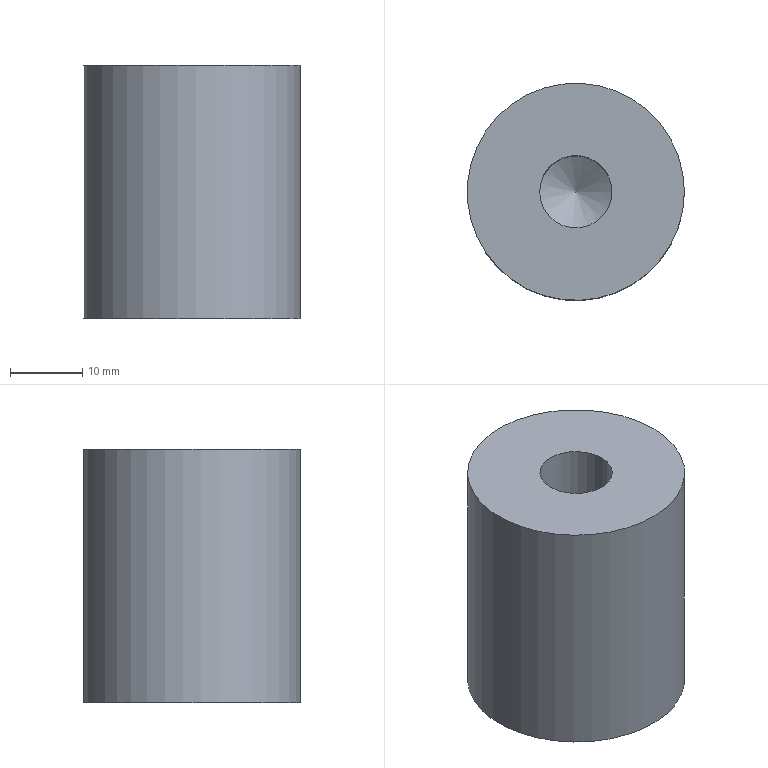Component | NX | CH3404_10-2 | 1 solid | 5 faces | box 30 x 30 x 35 mm | volume 22698 mm3 | cylinder 2 | plane 2 | cone 1 | commonest cylinder face diameters 30 x1 10 x1
STEP:
#1=CARTESIAN_POINT('',(0.,0.,0.));
#2=DIRECTION('',(0.,0.,1.));
#3=DIRECTION('',(1.,0.,0.));
#4=AXIS2_PLACEMENT_3D('',#1,#2,#3);
#5=CARTESIAN_POINT('',(15.,0.,146.));
#6=VERTEX_POINT('',#5);
#7=CARTESIAN_POINT('',(0.,0.,146.));
#8=DIRECTION('',(0.,0.,1.));
#9=DIRECTION('',(1.,0.,0.));
#10=AXIS2_PLACEMENT_3D('',#7,#8,#9);
#11=CIRCLE('',#10,15.);
#12=CARTESIAN_POINT('',(0.,0.,146.));
#13=DIRECTION('',(0.,0.,-1.));
#14=DIRECTION('',(-1.,0.,0.));
#15=AXIS2_PLACEMENT_3D('',#12,#13,#14);
#16=CYLINDRICAL_SURFACE('',#15,15.);
#17=CARTESIAN_POINT('',(9.425,0.));
#18=DIRECTION('',(-1.,0.));
#19=VECTOR('',#18,1.);
#20=LINE('',#17,#19);
#21=(GEOMETRIC_REPRESENTATION_CONTEXT(2)PARAMETRIC_REPRESENTATION_CONTEXT()REPRESENTATION_CONTEXT('',''));
#22=DEFINITIONAL_REPRESENTATION('',(#20),#21);
#23=PCURVE('',#16,#22);
#24=CARTESIAN_POINT('',(0.,0.,146.));
#25=DIRECTION('',(0.,0.,1.));
#26=DIRECTION('',(1.,0.,0.));
#27=AXIS2_PLACEMENT_3D('',#24,#25,#26);
#28=PLANE('',#27);
#29=CARTESIAN_POINT('',(0.,0.));
#30=DIRECTION('',(1.,0.));
#31=AXIS2_PLACEMENT_2D('',#29,#30);
#32=CIRCLE('',#31,15.);
#33=(GEOMETRIC_REPRESENTATION_CONTEXT(2)PARAMETRIC_REPRESENTATION_CONTEXT()REPRESENTATION_CONTEXT('',''));
#34=DEFINITIONAL_REPRESENTATION('',(#32),#33);
#35=PCURVE('',#28,#34);
#36=SURFACE_CURVE('',#11,(#23,#35),.PCURVE_S1.);
#37=EDGE_CURVE('',#6,#6,#36,.T.);
#38=ORIENTED_EDGE('',*,*,#37,.F.);
#39=CARTESIAN_POINT('',(15.,0.,111.));
#40=VERTEX_POINT('',#39);
#41=CARTESIAN_POINT('',(15.,0.,146.));
#42=CARTESIAN_POINT('',(15.,0.,111.));
#43=B_SPLINE_CURVE_WITH_KNOTS('',1,(#41,#42),.UNSPECIFIED.,.F.,.F.,(2,2),(0.,35.),.PIECEWISE_BEZIER_KNOTS.);
#44=CARTESIAN_POINT('',(9.425,0.));
#45=DIRECTION('',(0.,1.));
#46=VECTOR('',#45,1.);
#47=LINE('',#44,#46);
#48=(GEOMETRIC_REPRESENTATION_CONTEXT(2)PARAMETRIC_REPRESENTATION_CONTEXT()REPRESENTATION_CONTEXT('',''));
#49=DEFINITIONAL_REPRESENTATION('',(#47),#48);
#50=PCURVE('',#16,#49);
#51=CARTESIAN_POINT('',(3.142,0.));
#52=DIRECTION('',(0.,1.));
#53=VECTOR('',#52,1.);
#54=LINE('',#51,#53);
#55=(GEOMETRIC_REPRESENTATION_CONTEXT(2)PARAMETRIC_REPRESENTATION_CONTEXT()REPRESENTATION_CONTEXT('',''));
#56=DEFINITIONAL_REPRESENTATION('',(#54),#55);
#57=PCURVE('',#16,#56);
#58=SEAM_CURVE('',#43,(#50,#57),.PCURVE_S1.);
#59=EDGE_CURVE('',#6,#40,#58,.T.);
#60=ORIENTED_EDGE('',*,*,#59,.T.);
#61=CARTESIAN_POINT('',(0.,0.,111.));
#62=DIRECTION('',(0.,0.,1.));
#63=DIRECTION('',(1.,0.,0.));
#64=AXIS2_PLACEMENT_3D('',#61,#62,#63);
#65=CIRCLE('',#64,15.);
#66=CARTESIAN_POINT('',(9.425,35.));
#67=DIRECTION('',(-1.,0.));
#68=VECTOR('',#67,1.);
#69=LINE('',#66,#68);
#70=(GEOMETRIC_REPRESENTATION_CONTEXT(2)PARAMETRIC_REPRESENTATION_CONTEXT()REPRESENTATION_CONTEXT('',''));
#71=DEFINITIONAL_REPRESENTATION('',(#69),#70);
#72=PCURVE('',#16,#71);
#73=CARTESIAN_POINT('',(0.,0.,111.));
#74=DIRECTION('',(0.,0.,1.));
#75=DIRECTION('',(1.,0.,0.));
#76=AXIS2_PLACEMENT_3D('',#73,#74,#75);
#77=PLANE('',#76);
#78=CARTESIAN_POINT('',(0.,0.));
#79=DIRECTION('',(1.,0.));
#80=AXIS2_PLACEMENT_2D('',#78,#79);
#81=CIRCLE('',#80,15.);
#82=(GEOMETRIC_REPRESENTATION_CONTEXT(2)PARAMETRIC_REPRESENTATION_CONTEXT()REPRESENTATION_CONTEXT('',''));
#83=DEFINITIONAL_REPRESENTATION('',(#81),#82);
#84=PCURVE('',#77,#83);
#85=SURFACE_CURVE('',#65,(#72,#84),.PCURVE_S1.);
#86=EDGE_CURVE('',#40,#40,#85,.T.);
#87=ORIENTED_EDGE('',*,*,#86,.T.);
#88=ORIENTED_EDGE('',*,*,#59,.F.);
#89=EDGE_LOOP('',(#38,#60,#87,#88));
#90=FACE_BOUND('',#89,.T.);
#91=ADVANCED_FACE('',(#90),#16,.T.);
#92=CARTESIAN_POINT('',(-5.,0.,146.));
#93=VERTEX_POINT('',#92);
#94=CARTESIAN_POINT('',(0.,0.,146.));
#95=DIRECTION('',(0.,0.,-1.));
#96=DIRECTION('',(-1.,0.,0.));
#97=AXIS2_PLACEMENT_3D('',#94,#95,#96);
#98=CIRCLE('',#97,5.);
#99=CARTESIAN_POINT('',(-5.,0.));
#100=CARTESIAN_POINT('',(-5.,8.66));
#101=CARTESIAN_POINT('',(2.5,4.33));
#102=CARTESIAN_POINT('',(10.,0.));
#103=CARTESIAN_POINT('',(2.5,-4.33));
#104=CARTESIAN_POINT('',(-5.,-8.66));
#105=CARTESIAN_POINT('',(-5.,0.));
#106=(BOUNDED_CURVE()B_SPLINE_CURVE(2,(#99,#100,#101,#102,#103,#104,#105),.UNSPECIFIED.,.T.,.F.)B_SPLINE_CURVE_WITH_KNOTS((1,2,2,2,2,1),(-2.094,0.,2.094,4.189,6.283,8.378),.UNSPECIFIED.)CURVE()GEOMETRIC_REPRESENTATION_ITEM()RATIONAL_B_SPLINE_CURVE((1.,0.5,1.,0.5,1.,0.5,1.))REPRESENTATION_ITEM(''));
#107=(GEOMETRIC_REPRESENTATION_CONTEXT(2)PARAMETRIC_REPRESENTATION_CONTEXT()REPRESENTATION_CONTEXT('',''));
#108=DEFINITIONAL_REPRESENTATION('',(#106),#107);
#109=PCURVE('',#28,#108);
#110=CARTESIAN_POINT('',(0.,0.,146.));
#111=DIRECTION('',(0.,0.,-1.));
#112=DIRECTION('',(-1.,0.,0.));
#113=AXIS2_PLACEMENT_3D('',#110,#111,#112);
#114=CYLINDRICAL_SURFACE('',#113,5.);
#115=CARTESIAN_POINT('',(0.,0.));
#116=DIRECTION('',(1.,0.));
#117=VECTOR('',#116,1.);
#118=LINE('',#115,#117);
#119=(GEOMETRIC_REPRESENTATION_CONTEXT(2)PARAMETRIC_REPRESENTATION_CONTEXT()REPRESENTATION_CONTEXT('',''));
#120=DEFINITIONAL_REPRESENTATION('',(#118),#119);
#121=PCURVE('',#114,#120);
#122=SURFACE_CURVE('',#98,(#109,#121),.PCURVE_S1.);
#123=EDGE_CURVE('',#93,#93,#122,.T.);
#124=ORIENTED_EDGE('',*,*,#123,.T.);
#125=EDGE_LOOP('',(#124));
#126=FACE_BOUND('',#125,.T.);
#127=ORIENTED_EDGE('',*,*,#37,.T.);
#128=EDGE_LOOP('',(#127));
#129=FACE_BOUND('',#128,.T.);
#130=ADVANCED_FACE('',(#126,#129),#28,.T.);
#131=ORIENTED_EDGE('',*,*,#86,.F.);
#132=EDGE_LOOP('',(#131));
#133=FACE_BOUND('',#132,.T.);
#134=ADVANCED_FACE('',(#133),#77,.F.);
#135=CARTESIAN_POINT('',(-5.,0.,121.));
#136=VERTEX_POINT('',#135);
#137=CARTESIAN_POINT('',(5.,0.,121.));
#138=VERTEX_POINT('',#137);
#139=CARTESIAN_POINT('',(0.,0.,121.));
#140=DIRECTION('',(0.,0.,-1.));
#141=DIRECTION('',(-1.,0.,0.));
#142=AXIS2_PLACEMENT_3D('',#139,#140,#141);
#143=CIRCLE('',#142,5.);
#144=CARTESIAN_POINT('',(0.,0.,121.));
#145=DIRECTION('',(0.,0.,1.));
#146=DIRECTION('',(1.,0.,0.));
#147=AXIS2_PLACEMENT_3D('',#144,#145,#146);
#148=CONICAL_SURFACE('',#147,5.,1.03);
#149=CARTESIAN_POINT('',(3.142,0.));
#150=DIRECTION('',(-1.,0.));
#151=VECTOR('',#150,1.);
#152=LINE('',#149,#151);
#153=(GEOMETRIC_REPRESENTATION_CONTEXT(2)PARAMETRIC_REPRESENTATION_CONTEXT()REPRESENTATION_CONTEXT('',''));
#154=DEFINITIONAL_REPRESENTATION('',(#152),#153);
#155=PCURVE('',#148,#154);
#156=CARTESIAN_POINT('',(0.,25.));
#157=DIRECTION('',(1.,0.));
#158=VECTOR('',#157,1.);
#159=LINE('',#156,#158);
#160=(GEOMETRIC_REPRESENTATION_CONTEXT(2)PARAMETRIC_REPRESENTATION_CONTEXT()REPRESENTATION_CONTEXT('',''));
#161=DEFINITIONAL_REPRESENTATION('',(#159),#160);
#162=PCURVE('',#114,#161);
#163=SURFACE_CURVE('',#143,(#155,#162),.PCURVE_S1.);
#164=EDGE_CURVE('',#136,#138,#163,.T.);
#165=ORIENTED_EDGE('',*,*,#164,.T.);
#166=CARTESIAN_POINT('',(0.,0.,117.996));
#167=VERTEX_POINT('',#166);
#168=CARTESIAN_POINT('',(0.,-0.,117.996));
#169=CARTESIAN_POINT('',(5.,-0.,121.));
#170=B_SPLINE_CURVE_WITH_KNOTS('',1,(#168,#169),.UNSPECIFIED.,.F.,.F.,(2,2),(-5.833,0.),.PIECEWISE_BEZIER_KNOTS.);
#171=CARTESIAN_POINT('',(0.,0.));
#172=DIRECTION('',(0.,1.));
#173=VECTOR('',#172,1.);
#174=LINE('',#171,#173);
#175=(GEOMETRIC_REPRESENTATION_CONTEXT(2)PARAMETRIC_REPRESENTATION_CONTEXT()REPRESENTATION_CONTEXT('',''));
#176=DEFINITIONAL_REPRESENTATION('',(#174),#175);
#177=PCURVE('',#148,#176);
#178=CARTESIAN_POINT('',(6.283,0.));
#179=DIRECTION('',(0.,1.));
#180=VECTOR('',#179,1.);
#181=LINE('',#178,#180);
#182=(GEOMETRIC_REPRESENTATION_CONTEXT(2)PARAMETRIC_REPRESENTATION_CONTEXT()REPRESENTATION_CONTEXT('',''));
#183=DEFINITIONAL_REPRESENTATION('',(#181),#182);
#184=PCURVE('',#148,#183);
#185=SEAM_CURVE('',#170,(#177,#184),.PCURVE_S1.);
#186=EDGE_CURVE('',#167,#138,#185,.T.);
#187=ORIENTED_EDGE('',*,*,#186,.F.);
#188=ORIENTED_EDGE('',*,*,#186,.T.);
#189=CARTESIAN_POINT('',(0.,0.,121.));
#190=DIRECTION('',(0.,0.,-1.));
#191=DIRECTION('',(-1.,0.,0.));
#192=AXIS2_PLACEMENT_3D('',#189,#190,#191);
#193=CIRCLE('',#192,5.);
#194=CARTESIAN_POINT('',(9.425,0.));
#195=DIRECTION('',(-1.,0.));
#196=VECTOR('',#195,1.);
#197=LINE('',#194,#196);
#198=(GEOMETRIC_REPRESENTATION_CONTEXT(2)PARAMETRIC_REPRESENTATION_CONTEXT()REPRESENTATION_CONTEXT('',''));
#199=DEFINITIONAL_REPRESENTATION('',(#197),#198);
#200=PCURVE('',#148,#199);
#201=CARTESIAN_POINT('',(0.,25.));
#202=DIRECTION('',(1.,0.));
#203=VECTOR('',#202,1.);
#204=LINE('',#201,#203);
#205=(GEOMETRIC_REPRESENTATION_CONTEXT(2)PARAMETRIC_REPRESENTATION_CONTEXT()REPRESENTATION_CONTEXT('',''));
#206=DEFINITIONAL_REPRESENTATION('',(#204),#205);
#207=PCURVE('',#114,#206);
#208=SURFACE_CURVE('',#193,(#200,#207),.PCURVE_S1.);
#209=EDGE_CURVE('',#138,#136,#208,.T.);
#210=ORIENTED_EDGE('',*,*,#209,.T.);
#211=EDGE_LOOP('',(#165,#187,#188,#210));
#212=FACE_BOUND('',#211,.F.);
#213=ADVANCED_FACE('',(#212),#148,.F.);
#214=ORIENTED_EDGE('',*,*,#209,.F.);
#215=ORIENTED_EDGE('',*,*,#164,.F.);
#216=CARTESIAN_POINT('',(-5.,-0.,146.));
#217=CARTESIAN_POINT('',(-5.,-0.,121.));
#218=B_SPLINE_CURVE_WITH_KNOTS('',1,(#216,#217),.UNSPECIFIED.,.F.,.F.,(2,2),(0.,25.),.PIECEWISE_BEZIER_KNOTS.);
#219=CARTESIAN_POINT('',(0.,0.));
#220=DIRECTION('',(0.,1.));
#221=VECTOR('',#220,1.);
#222=LINE('',#219,#221);
#223=(GEOMETRIC_REPRESENTATION_CONTEXT(2)PARAMETRIC_REPRESENTATION_CONTEXT()REPRESENTATION_CONTEXT('',''));
#224=DEFINITIONAL_REPRESENTATION('',(#222),#223);
#225=PCURVE('',#114,#224);
#226=CARTESIAN_POINT('',(6.283,0.));
#227=DIRECTION('',(0.,1.));
#228=VECTOR('',#227,1.);
#229=LINE('',#226,#228);
#230=(GEOMETRIC_REPRESENTATION_CONTEXT(2)PARAMETRIC_REPRESENTATION_CONTEXT()REPRESENTATION_CONTEXT('',''));
#231=DEFINITIONAL_REPRESENTATION('',(#229),#230);
#232=PCURVE('',#114,#231);
#233=SEAM_CURVE('',#218,(#225,#232),.PCURVE_S1.);
#234=EDGE_CURVE('',#93,#136,#233,.T.);
#235=ORIENTED_EDGE('',*,*,#234,.F.);
#236=ORIENTED_EDGE('',*,*,#123,.T.);
#237=ORIENTED_EDGE('',*,*,#234,.T.);
#238=EDGE_LOOP('',(#214,#215,#235,#236,#237));
#239=FACE_BOUND('',#238,.F.);
#240=ADVANCED_FACE('',(#239),#114,.F.);
#241=CLOSED_SHELL('',(#91,#130,#134,#213,#240));
#242=MANIFOLD_SOLID_BREP('',#241);
#243=(LENGTH_UNIT()NAMED_UNIT(*)SI_UNIT(.MILLI.,.METRE.));
#244=UNCERTAINTY_MEASURE_WITH_UNIT(LENGTH_MEASURE(0.00001),#243,'','');
#245=(NAMED_UNIT(*)PLANE_ANGLE_UNIT()SI_UNIT($,.RADIAN.));
#246=(NAMED_UNIT(*)SI_UNIT($,.STERADIAN.)SOLID_ANGLE_UNIT());
#247=(GEOMETRIC_REPRESENTATION_CONTEXT(3)GLOBAL_UNCERTAINTY_ASSIGNED_CONTEXT((#244))GLOBAL_UNIT_ASSIGNED_CONTEXT((#243,#245,#246))REPRESENTATION_CONTEXT('',''));
#248=ADVANCED_BREP_SHAPE_REPRESENTATION('',(#4,#242),#247);